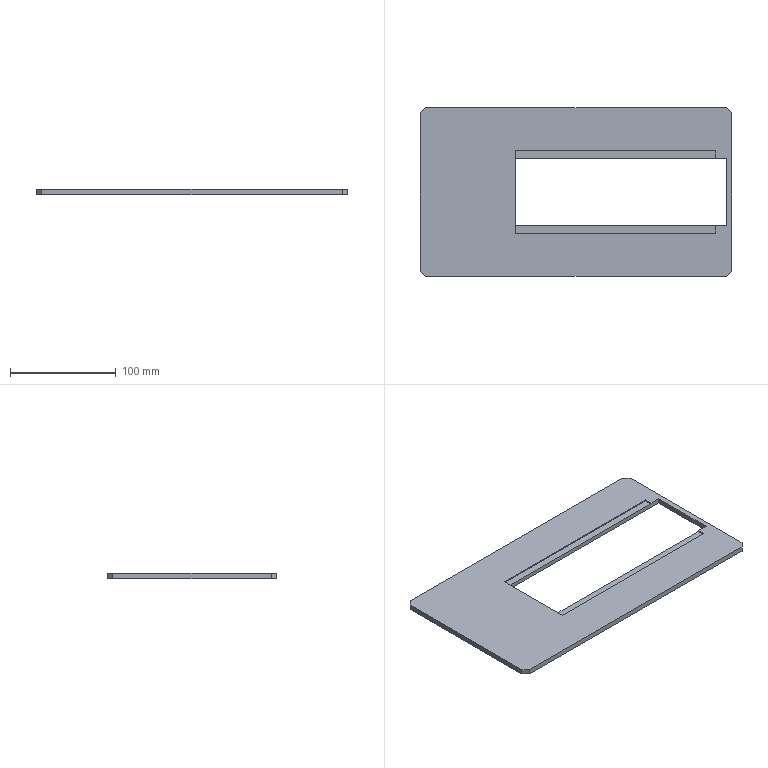Component | SolidWorks | 2023-12-12-25-1 | 1 solid | 38 faces | box 295 x 160 x 5 mm | volume 166969 mm3 | plane 26 | cylinder 12 | commonest cylinder face diameters 15 x12 | material S45C
build123d program:
from build123d import *

# Parameters (mm, degrees)
SKETCH1_2_W          = 200
SKETCH1_2_H          = 64
BOSS_EXTRUDE1_DEPTH  = 5
SKETCH3_R            = 7.5
CUT_EXTRUDE2_DEPTH   = 2
CHAMFER2_SIZE        = 5
SKETCH4_W            = 25
SKETCH4_H            = 160
CUT_EXTRUDE3_DEPTH   = 10
CHAMFER3_SIZE        = 5
SKETCH1_W            = 190
SKETCH1_H            = 8
RAILSEATREBATE_DEPTH = 1


with BuildPart() as part:
    # Sketch1_2 → Boss-Extrude1 (new body)
    with BuildSketch(Plane.XY):
        Polygon((0, 0), (320, 0), (320, 18), (320, 160), (0, 160), align=None)
        with Locations((130, 80)):
            Rectangle(SKETCH1_2_W, SKETCH1_2_H, mode=Mode.SUBTRACT)
    extrude(amount=BOSS_EXTRUDE1_DEPTH)

    # Sketch3 → Cut-Extrude2 (cut)
    with BuildSketch(Plane(origin=(0, 0, 0), x_dir=(-1, 0, 0), z_dir=(0, 0, -1))):
        with Locations((-305, 150)):
            Circle(SKETCH3_R)
        with Locations((-105, 150)):
            Circle(SKETCH3_R)
        with Locations((-40, 150)):
            Circle(SKETCH3_R)
        with Locations(Location((-40, 10, 0), (0, 0, 180))):
            Circle(SKETCH3_R)
        with Locations(Location((-105, 10, 0), (0, 0, 180))):
            Circle(SKETCH3_R)
        with Locations(Location((-305, 10, 0), (0, 0, 180))):
            Circle(SKETCH3_R)
    extrude(amount=-CUT_EXTRUDE2_DEPTH, mode=Mode.SUBTRACT)

    # Chamfer2
    chamfer2_edges = [part.edges().sort_by_distance(p)[0] for p in [
        (0, 160, 2.5),
        (320, 160, 2.5),
        (320, 0, 2.5),
        (0, 0, 2.5),
    ]]
    chamfer(chamfer2_edges, length=CHAMFER2_SIZE)

    # Sketch4 → Cut-Extrude3 (cut)
    with BuildSketch(Plane(origin=(0, 0, 0), x_dir=(-1, 0, 0), z_dir=(0, 0, -1))):
        with Locations((-12.5, 80)):
            Rectangle(SKETCH4_W, SKETCH4_H)
    extrude(amount=-CUT_EXTRUDE3_DEPTH, mode=Mode.SUBTRACT)

    # Chamfer3
    chamfer3_edges = [part.edges().sort_by_distance(p)[0] for p in [
        (25, 0, 2.5),
        (25, 160, 2.5),
    ]]
    chamfer(chamfer3_edges, length=CHAMFER3_SIZE)

    # Sketch1 → RailSeatRebate (cut)
    with BuildSketch(Plane.XY.offset(5)):
        with Locations((135, 45)):
            Rectangle(SKETCH1_W, SKETCH1_H)
        with Locations((135, 115)):
            Rectangle(SKETCH1_W, SKETCH1_H)
    extrude(amount=-RAILSEATREBATE_DEPTH, mode=Mode.SUBTRACT)


solid = part.part

# Placed as in the assembly
solid = solid.moved(Location((131.222, 77.133, 79), (0, 0, 180)))
STEP:
#1=COLOUR_RGB('',0.7922,0.8196,0.9333);
#2=FILL_AREA_STYLE_COLOUR('',#1);
#3=FILL_AREA_STYLE('',(#2));
#4=SURFACE_STYLE_FILL_AREA(#3);
#5=SURFACE_SIDE_STYLE('',(#4));
#6=SURFACE_STYLE_USAGE(.BOTH.,#5);
#7=PRESENTATION_STYLE_ASSIGNMENT((#6));
#8=CARTESIAN_POINT('',(3.296,-2.869,3.189));
#9=VERTEX_POINT('',#8);
#10=CARTESIAN_POINT('',(3.887,-2.869,3.189));
#11=VERTEX_POINT('',#10);
#12=CARTESIAN_POINT('',(3.591,-2.869,3.189));
#13=DIRECTION('',(0.,0.,-1.));
#14=DIRECTION('',(1.,0.,0.));
#15=AXIS2_PLACEMENT_3D('',#12,#13,#14);
#16=CIRCLE('',#15,0.2953);
#17=EDGE_CURVE('',#9,#11,#16,.T.);
#18=ORIENTED_EDGE('',*,*,#17,.F.);
#19=CARTESIAN_POINT('',(3.296,-2.869,3.11));
#20=VERTEX_POINT('',#19);
#21=CARTESIAN_POINT('',(3.296,-2.869,3.189));
#22=DIRECTION('',(0.,0.,-1.));
#23=VECTOR('',#22,39.37);
#24=LINE('',#21,#23);
#25=EDGE_CURVE('',#9,#20,#24,.T.);
#26=ORIENTED_EDGE('',*,*,#25,.T.);
#27=CARTESIAN_POINT('',(3.887,-2.869,3.11));
#28=VERTEX_POINT('',#27);
#29=CARTESIAN_POINT('',(3.591,-2.869,3.11));
#30=DIRECTION('',(0.,0.,-1.));
#31=DIRECTION('',(1.,0.,0.));
#32=AXIS2_PLACEMENT_3D('',#29,#30,#31);
#33=CIRCLE('',#32,0.2953);
#34=EDGE_CURVE('',#20,#28,#33,.T.);
#35=ORIENTED_EDGE('',*,*,#34,.T.);
#36=CARTESIAN_POINT('',(3.887,-2.869,3.189));
#37=DIRECTION('',(0.,0.,-1.));
#38=VECTOR('',#37,39.37);
#39=LINE('',#36,#38);
#40=EDGE_CURVE('',#11,#28,#39,.T.);
#41=ORIENTED_EDGE('',*,*,#40,.F.);
#42=EDGE_LOOP('',(#18,#26,#35,#41));
#43=FACE_OUTER_BOUND('',#42,.T.);
#44=CARTESIAN_POINT('',(3.591,-2.869,3.189));
#45=DIRECTION('',(0.,0.,-1.));
#46=DIRECTION('',(1.,0.,0.));
#47=AXIS2_PLACEMENT_3D('',#44,#45,#46);
#48=CYLINDRICAL_SURFACE('',#47,0.2953);
#49=ADVANCED_FACE('',(#43),#48,.F.);
#50=CARTESIAN_POINT('',(-7.137,-2.869,3.189));
#51=VERTEX_POINT('',#50);
#52=CARTESIAN_POINT('',(-6.546,-2.869,3.189));
#53=VERTEX_POINT('',#52);
#54=CARTESIAN_POINT('',(-6.842,-2.869,3.189));
#55=DIRECTION('',(0.,0.,-1.));
#56=DIRECTION('',(1.,0.,0.));
#57=AXIS2_PLACEMENT_3D('',#54,#55,#56);
#58=CIRCLE('',#57,0.2953);
#59=EDGE_CURVE('',#51,#53,#58,.T.);
#60=ORIENTED_EDGE('',*,*,#59,.F.);
#61=CARTESIAN_POINT('',(-7.137,-2.869,3.11));
#62=VERTEX_POINT('',#61);
#63=CARTESIAN_POINT('',(-7.137,-2.869,3.189));
#64=DIRECTION('',(0.,0.,-1.));
#65=VECTOR('',#64,39.37);
#66=LINE('',#63,#65);
#67=EDGE_CURVE('',#51,#62,#66,.T.);
#68=ORIENTED_EDGE('',*,*,#67,.T.);
#69=CARTESIAN_POINT('',(-6.546,-2.869,3.11));
#70=VERTEX_POINT('',#69);
#71=CARTESIAN_POINT('',(-6.842,-2.869,3.11));
#72=DIRECTION('',(0.,0.,-1.));
#73=DIRECTION('',(1.,0.,0.));
#74=AXIS2_PLACEMENT_3D('',#71,#72,#73);
#75=CIRCLE('',#74,0.2953);
#76=EDGE_CURVE('',#62,#70,#75,.T.);
#77=ORIENTED_EDGE('',*,*,#76,.T.);
#78=CARTESIAN_POINT('',(-6.546,-2.869,3.189));
#79=DIRECTION('',(0.,0.,-1.));
#80=VECTOR('',#79,39.37);
#81=LINE('',#78,#80);
#82=EDGE_CURVE('',#53,#70,#81,.T.);
#83=ORIENTED_EDGE('',*,*,#82,.F.);
#84=EDGE_LOOP('',(#60,#68,#77,#83));
#85=FACE_OUTER_BOUND('',#84,.T.);
#86=CARTESIAN_POINT('',(-6.842,-2.869,3.189));
#87=DIRECTION('',(0.,0.,-1.));
#88=DIRECTION('',(1.,0.,0.));
#89=AXIS2_PLACEMENT_3D('',#86,#87,#88);
#90=CYLINDRICAL_SURFACE('',#89,0.2953);
#91=ADVANCED_FACE('',(#85),#90,.F.);
#92=CARTESIAN_POINT('',(3.296,2.643,3.189));
#93=VERTEX_POINT('',#92);
#94=CARTESIAN_POINT('',(3.887,2.643,3.189));
#95=VERTEX_POINT('',#94);
#96=CARTESIAN_POINT('',(3.591,2.643,3.189));
#97=DIRECTION('',(0.,0.,-1.));
#98=DIRECTION('',(-1.,0.,0.));
#99=AXIS2_PLACEMENT_3D('',#96,#97,#98);
#100=CIRCLE('',#99,0.2953);
#101=EDGE_CURVE('',#93,#95,#100,.T.);
#102=ORIENTED_EDGE('',*,*,#101,.F.);
#103=CARTESIAN_POINT('',(3.296,2.643,3.11));
#104=VERTEX_POINT('',#103);
#105=CARTESIAN_POINT('',(3.296,2.643,3.189));
#106=DIRECTION('',(0.,0.,-1.));
#107=VECTOR('',#106,39.37);
#108=LINE('',#105,#107);
#109=EDGE_CURVE('',#93,#104,#108,.T.);
#110=ORIENTED_EDGE('',*,*,#109,.T.);
#111=CARTESIAN_POINT('',(3.887,2.643,3.11));
#112=VERTEX_POINT('',#111);
#113=CARTESIAN_POINT('',(3.591,2.643,3.11));
#114=DIRECTION('',(0.,0.,-1.));
#115=DIRECTION('',(-1.,0.,0.));
#116=AXIS2_PLACEMENT_3D('',#113,#114,#115);
#117=CIRCLE('',#116,0.2953);
#118=EDGE_CURVE('',#104,#112,#117,.T.);
#119=ORIENTED_EDGE('',*,*,#118,.T.);
#120=CARTESIAN_POINT('',(3.887,2.643,3.189));
#121=DIRECTION('',(0.,0.,-1.));
#122=VECTOR('',#121,39.37);
#123=LINE('',#120,#122);
#124=EDGE_CURVE('',#95,#112,#123,.T.);
#125=ORIENTED_EDGE('',*,*,#124,.F.);
#126=EDGE_LOOP('',(#102,#110,#119,#125));
#127=FACE_OUTER_BOUND('',#126,.T.);
#128=CARTESIAN_POINT('',(3.591,2.643,3.189));
#129=DIRECTION('',(0.,0.,-1.));
#130=DIRECTION('',(1.,0.,0.));
#131=AXIS2_PLACEMENT_3D('',#128,#129,#130);
#132=CYLINDRICAL_SURFACE('',#131,0.2953);
#133=ADVANCED_FACE('',(#127),#132,.F.);
#134=CARTESIAN_POINT('',(0.7371,2.643,3.189));
#135=VERTEX_POINT('',#134);
#136=CARTESIAN_POINT('',(1.328,2.643,3.189));
#137=VERTEX_POINT('',#136);
#138=CARTESIAN_POINT('',(1.032,2.643,3.189));
#139=DIRECTION('',(0.,0.,-1.));
#140=DIRECTION('',(-1.,0.,0.));
#141=AXIS2_PLACEMENT_3D('',#138,#139,#140);
#142=CIRCLE('',#141,0.2953);
#143=EDGE_CURVE('',#135,#137,#142,.T.);
#144=ORIENTED_EDGE('',*,*,#143,.F.);
#145=CARTESIAN_POINT('',(0.7371,2.643,3.11));
#146=VERTEX_POINT('',#145);
#147=CARTESIAN_POINT('',(0.7371,2.643,3.189));
#148=DIRECTION('',(0.,0.,-1.));
#149=VECTOR('',#148,39.37);
#150=LINE('',#147,#149);
#151=EDGE_CURVE('',#135,#146,#150,.T.);
#152=ORIENTED_EDGE('',*,*,#151,.T.);
#153=CARTESIAN_POINT('',(1.328,2.643,3.11));
#154=VERTEX_POINT('',#153);
#155=CARTESIAN_POINT('',(1.032,2.643,3.11));
#156=DIRECTION('',(0.,0.,-1.));
#157=DIRECTION('',(-1.,0.,0.));
#158=AXIS2_PLACEMENT_3D('',#155,#156,#157);
#159=CIRCLE('',#158,0.2953);
#160=EDGE_CURVE('',#146,#154,#159,.T.);
#161=ORIENTED_EDGE('',*,*,#160,.T.);
#162=CARTESIAN_POINT('',(1.328,2.643,3.189));
#163=DIRECTION('',(0.,0.,-1.));
#164=VECTOR('',#163,39.37);
#165=LINE('',#162,#164);
#166=EDGE_CURVE('',#137,#154,#165,.T.);
#167=ORIENTED_EDGE('',*,*,#166,.F.);
#168=EDGE_LOOP('',(#144,#152,#161,#167));
#169=FACE_OUTER_BOUND('',#168,.T.);
#170=CARTESIAN_POINT('',(1.032,2.643,3.189));
#171=DIRECTION('',(0.,0.,-1.));
#172=DIRECTION('',(1.,0.,0.));
#173=AXIS2_PLACEMENT_3D('',#170,#171,#172);
#174=CYLINDRICAL_SURFACE('',#173,0.2953);
#175=ADVANCED_FACE('',(#169),#174,.F.);
#176=CARTESIAN_POINT('',(-7.137,2.643,3.189));
#177=VERTEX_POINT('',#176);
#178=CARTESIAN_POINT('',(-6.546,2.643,3.189));
#179=VERTEX_POINT('',#178);
#180=CARTESIAN_POINT('',(-6.842,2.643,3.189));
#181=DIRECTION('',(0.,0.,-1.));
#182=DIRECTION('',(-1.,0.,0.));
#183=AXIS2_PLACEMENT_3D('',#180,#181,#182);
#184=CIRCLE('',#183,0.2953);
#185=EDGE_CURVE('',#177,#179,#184,.T.);
#186=ORIENTED_EDGE('',*,*,#185,.F.);
#187=CARTESIAN_POINT('',(-7.137,2.643,3.11));
#188=VERTEX_POINT('',#187);
#189=CARTESIAN_POINT('',(-7.137,2.643,3.189));
#190=DIRECTION('',(0.,0.,-1.));
#191=VECTOR('',#190,39.37);
#192=LINE('',#189,#191);
#193=EDGE_CURVE('',#177,#188,#192,.T.);
#194=ORIENTED_EDGE('',*,*,#193,.T.);
#195=CARTESIAN_POINT('',(-6.546,2.643,3.11));
#196=VERTEX_POINT('',#195);
#197=CARTESIAN_POINT('',(-6.842,2.643,3.11));
#198=DIRECTION('',(0.,0.,-1.));
#199=DIRECTION('',(-1.,0.,0.));
#200=AXIS2_PLACEMENT_3D('',#197,#198,#199);
#201=CIRCLE('',#200,0.2953);
#202=EDGE_CURVE('',#188,#196,#201,.T.);
#203=ORIENTED_EDGE('',*,*,#202,.T.);
#204=CARTESIAN_POINT('',(-6.546,2.643,3.189));
#205=DIRECTION('',(0.,0.,-1.));
#206=VECTOR('',#205,39.37);
#207=LINE('',#204,#206);
#208=EDGE_CURVE('',#179,#196,#207,.T.);
#209=ORIENTED_EDGE('',*,*,#208,.F.);
#210=EDGE_LOOP('',(#186,#194,#203,#209));
#211=FACE_OUTER_BOUND('',#210,.T.);
#212=CARTESIAN_POINT('',(-6.842,2.643,3.189));
#213=DIRECTION('',(0.,0.,-1.));
#214=DIRECTION('',(1.,0.,0.));
#215=AXIS2_PLACEMENT_3D('',#212,#213,#214);
#216=CYLINDRICAL_SURFACE('',#215,0.2953);
#217=ADVANCED_FACE('',(#211),#216,.F.);
#218=CARTESIAN_POINT('',(0.7371,-2.869,3.189));
#219=VERTEX_POINT('',#218);
#220=CARTESIAN_POINT('',(1.328,-2.869,3.189));
#221=VERTEX_POINT('',#220);
#222=CARTESIAN_POINT('',(1.032,-2.869,3.189));
#223=DIRECTION('',(0.,0.,-1.));
#224=DIRECTION('',(1.,0.,0.));
#225=AXIS2_PLACEMENT_3D('',#222,#223,#224);
#226=CIRCLE('',#225,0.2953);
#227=EDGE_CURVE('',#219,#221,#226,.T.);
#228=ORIENTED_EDGE('',*,*,#227,.F.);
#229=CARTESIAN_POINT('',(0.7371,-2.869,3.11));
#230=VERTEX_POINT('',#229);
#231=CARTESIAN_POINT('',(0.7371,-2.869,3.189));
#232=DIRECTION('',(0.,0.,-1.));
#233=VECTOR('',#232,39.37);
#234=LINE('',#231,#233);
#235=EDGE_CURVE('',#219,#230,#234,.T.);
#236=ORIENTED_EDGE('',*,*,#235,.T.);
#237=CARTESIAN_POINT('',(1.328,-2.869,3.11));
#238=VERTEX_POINT('',#237);
#239=CARTESIAN_POINT('',(1.032,-2.869,3.11));
#240=DIRECTION('',(0.,0.,-1.));
#241=DIRECTION('',(1.,0.,0.));
#242=AXIS2_PLACEMENT_3D('',#239,#240,#241);
#243=CIRCLE('',#242,0.2953);
#244=EDGE_CURVE('',#230,#238,#243,.T.);
#245=ORIENTED_EDGE('',*,*,#244,.T.);
#246=CARTESIAN_POINT('',(1.328,-2.869,3.189));
#247=DIRECTION('',(0.,0.,-1.));
#248=VECTOR('',#247,39.37);
#249=LINE('',#246,#248);
#250=EDGE_CURVE('',#221,#238,#249,.T.);
#251=ORIENTED_EDGE('',*,*,#250,.F.);
#252=EDGE_LOOP('',(#228,#236,#245,#251));
#253=FACE_OUTER_BOUND('',#252,.T.);
#254=CARTESIAN_POINT('',(1.032,-2.869,3.189));
#255=DIRECTION('',(0.,0.,-1.));
#256=DIRECTION('',(1.,0.,0.));
#257=AXIS2_PLACEMENT_3D('',#254,#255,#256);
#258=CYLINDRICAL_SURFACE('',#257,0.2953);
#259=ADVANCED_FACE('',(#253),#258,.F.);
#260=CARTESIAN_POINT('',(-7.235,-3.262,3.307));
#261=VERTEX_POINT('',#260);
#262=CARTESIAN_POINT('',(3.985,-3.262,3.307));
#263=VERTEX_POINT('',#262);
#264=CARTESIAN_POINT('',(5.166,-3.262,3.307));
#265=DIRECTION('',(1.,0.,0.));
#266=VECTOR('',#265,39.37);
#267=LINE('',#264,#266);
#268=EDGE_CURVE('',#261,#263,#267,.T.);
#269=ORIENTED_EDGE('',*,*,#268,.T.);
#270=CARTESIAN_POINT('',(4.182,-3.066,3.307));
#271=VERTEX_POINT('',#270);
#272=CARTESIAN_POINT('',(4.182,-3.066,3.307));
#273=DIRECTION('',(0.7071,0.7071,0.));
#274=VECTOR('',#273,39.37);
#275=LINE('',#272,#274);
#276=EDGE_CURVE('',#263,#271,#275,.T.);
#277=ORIENTED_EDGE('',*,*,#276,.T.);
#278=CARTESIAN_POINT('',(4.182,2.84,3.307));
#279=VERTEX_POINT('',#278);
#280=CARTESIAN_POINT('',(4.182,3.037,3.307));
#281=DIRECTION('',(0.,1.,0.));
#282=VECTOR('',#281,39.37);
#283=LINE('',#280,#282);
#284=EDGE_CURVE('',#271,#279,#283,.T.);
#285=ORIENTED_EDGE('',*,*,#284,.T.);
#286=CARTESIAN_POINT('',(3.985,3.037,3.307));
#287=VERTEX_POINT('',#286);
#288=CARTESIAN_POINT('',(3.985,3.037,3.307));
#289=DIRECTION('',(-0.7071,0.7071,0.));
#290=VECTOR('',#289,39.37);
#291=LINE('',#288,#290);
#292=EDGE_CURVE('',#279,#287,#291,.T.);
#293=ORIENTED_EDGE('',*,*,#292,.T.);
#294=CARTESIAN_POINT('',(-7.235,3.037,3.307));
#295=VERTEX_POINT('',#294);
#296=CARTESIAN_POINT('',(5.166,3.037,3.307));
#297=DIRECTION('',(-1.,0.,-0.));
#298=VECTOR('',#297,39.37);
#299=LINE('',#296,#298);
#300=EDGE_CURVE('',#287,#295,#299,.T.);
#301=ORIENTED_EDGE('',*,*,#300,.T.);
#302=CARTESIAN_POINT('',(-7.432,2.84,3.307));
#303=VERTEX_POINT('',#302);
#304=CARTESIAN_POINT('',(-7.432,2.84,3.307));
#305=DIRECTION('',(-0.7071,-0.7071,-0.));
#306=VECTOR('',#305,39.37);
#307=LINE('',#304,#306);
#308=EDGE_CURVE('',#295,#303,#307,.T.);
#309=ORIENTED_EDGE('',*,*,#308,.T.);
#310=CARTESIAN_POINT('',(-7.432,-3.066,3.307));
#311=VERTEX_POINT('',#310);
#312=CARTESIAN_POINT('',(-7.432,3.037,3.307));
#313=DIRECTION('',(-0.,-1.,-0.));
#314=VECTOR('',#313,39.37);
#315=LINE('',#312,#314);
#316=EDGE_CURVE('',#303,#311,#315,.T.);
#317=ORIENTED_EDGE('',*,*,#316,.T.);
#318=CARTESIAN_POINT('',(-7.235,-3.262,3.307));
#319=DIRECTION('',(0.7071,-0.7071,-0.));
#320=VECTOR('',#319,39.37);
#321=LINE('',#318,#320);
#322=EDGE_CURVE('',#311,#261,#321,.T.);
#323=ORIENTED_EDGE('',*,*,#322,.T.);
#324=EDGE_LOOP('',(#269,#277,#285,#293,#301,#309,#317,#323));
#325=FACE_OUTER_BOUND('',#324,.T.);
#326=CARTESIAN_POINT('',(3.591,1.147,3.307));
#327=VERTEX_POINT('',#326);
#328=CARTESIAN_POINT('',(3.591,1.423,3.307));
#329=VERTEX_POINT('',#328);
#330=CARTESIAN_POINT('',(3.591,1.423,3.307));
#331=DIRECTION('',(0.,1.,0.));
#332=VECTOR('',#331,39.37);
#333=LINE('',#330,#332);
#334=EDGE_CURVE('',#327,#329,#333,.T.);
#335=ORIENTED_EDGE('',*,*,#334,.F.);
#336=CARTESIAN_POINT('',(3.985,1.147,3.307));
#337=VERTEX_POINT('',#336);
#338=CARTESIAN_POINT('',(3.985,1.147,3.307));
#339=DIRECTION('',(-1.,0.,-0.));
#340=VECTOR('',#339,39.37);
#341=LINE('',#338,#340);
#342=EDGE_CURVE('',#337,#327,#341,.T.);
#343=ORIENTED_EDGE('',*,*,#342,.F.);
#344=CARTESIAN_POINT('',(3.985,-1.373,3.307));
#345=VERTEX_POINT('',#344);
#346=CARTESIAN_POINT('',(3.985,1.147,3.307));
#347=DIRECTION('',(0.,1.,0.));
#348=VECTOR('',#347,39.37);
#349=LINE('',#346,#348);
#350=EDGE_CURVE('',#345,#337,#349,.T.);
#351=ORIENTED_EDGE('',*,*,#350,.F.);
#352=CARTESIAN_POINT('',(3.591,-1.373,3.307));
#353=VERTEX_POINT('',#352);
#354=CARTESIAN_POINT('',(3.985,-1.373,3.307));
#355=DIRECTION('',(1.,-0.,0.));
#356=VECTOR('',#355,39.37);
#357=LINE('',#354,#356);
#358=EDGE_CURVE('',#353,#345,#357,.T.);
#359=ORIENTED_EDGE('',*,*,#358,.F.);
#360=CARTESIAN_POINT('',(3.591,-1.648,3.307));
#361=VERTEX_POINT('',#360);
#362=CARTESIAN_POINT('',(3.591,-1.333,3.307));
#363=DIRECTION('',(0.,1.,0.));
#364=VECTOR('',#363,39.37);
#365=LINE('',#362,#364);
#366=EDGE_CURVE('',#361,#353,#365,.T.);
#367=ORIENTED_EDGE('',*,*,#366,.F.);
#368=CARTESIAN_POINT('',(-3.889,-1.648,3.307));
#369=VERTEX_POINT('',#368);
#370=CARTESIAN_POINT('',(3.591,-1.648,3.307));
#371=DIRECTION('',(1.,-0.,0.));
#372=VECTOR('',#371,39.37);
#373=LINE('',#370,#372);
#374=EDGE_CURVE('',#369,#361,#373,.T.);
#375=ORIENTED_EDGE('',*,*,#374,.F.);
#376=CARTESIAN_POINT('',(-3.889,1.423,3.307));
#377=VERTEX_POINT('',#376);
#378=CARTESIAN_POINT('',(-3.889,-1.373,3.307));
#379=DIRECTION('',(-0.,-1.,-0.));
#380=VECTOR('',#379,39.37);
#381=LINE('',#378,#380);
#382=EDGE_CURVE('',#377,#369,#381,.T.);
#383=ORIENTED_EDGE('',*,*,#382,.F.);
#384=CARTESIAN_POINT('',(3.591,1.423,3.307));
#385=DIRECTION('',(-1.,0.,-0.));
#386=VECTOR('',#385,39.37);
#387=LINE('',#384,#386);
#388=EDGE_CURVE('',#329,#377,#387,.T.);
#389=ORIENTED_EDGE('',*,*,#388,.F.);
#390=EDGE_LOOP('',(#335,#343,#351,#359,#367,#375,#383,#389));
#391=FACE_BOUND('',#390,.T.);
#392=CARTESIAN_POINT('',(5.166,3.037,3.307));
#393=DIRECTION('',(0.,0.,-1.));
#394=DIRECTION('',(1.,-0.,0.));
#395=AXIS2_PLACEMENT_3D('',#392,#393,#394);
#396=PLANE('',#395);
#397=ADVANCED_FACE('',(#325,#391),#396,.F.);
#398=CARTESIAN_POINT('',(4.182,-3.066,3.11));
#399=VERTEX_POINT('',#398);
#400=CARTESIAN_POINT('',(4.182,2.84,3.11));
#401=VERTEX_POINT('',#400);
#402=CARTESIAN_POINT('',(4.182,-3.262,3.11));
#403=DIRECTION('',(0.,1.,0.));
#404=VECTOR('',#403,39.37);
#405=LINE('',#402,#404);
#406=EDGE_CURVE('',#399,#401,#405,.T.);
#407=ORIENTED_EDGE('',*,*,#406,.F.);
#408=CARTESIAN_POINT('',(3.985,-3.262,3.11));
#409=VERTEX_POINT('',#408);
#410=CARTESIAN_POINT('',(7.725,0.4777,3.11));
#411=DIRECTION('',(-0.7071,-0.7071,-0.));
#412=VECTOR('',#411,39.37);
#413=LINE('',#410,#412);
#414=EDGE_CURVE('',#399,#409,#413,.T.);
#415=ORIENTED_EDGE('',*,*,#414,.T.);
#416=CARTESIAN_POINT('',(-7.235,-3.262,3.11));
#417=VERTEX_POINT('',#416);
#418=CARTESIAN_POINT('',(5.166,-3.262,3.11));
#419=DIRECTION('',(1.,0.,0.));
#420=VECTOR('',#419,39.37);
#421=LINE('',#418,#420);
#422=EDGE_CURVE('',#417,#409,#421,.T.);
#423=ORIENTED_EDGE('',*,*,#422,.F.);
#424=CARTESIAN_POINT('',(-7.432,-3.066,3.11));
#425=VERTEX_POINT('',#424);
#426=CARTESIAN_POINT('',(-4.184,-6.314,3.11));
#427=DIRECTION('',(-0.7071,0.7071,0.));
#428=VECTOR('',#427,39.37);
#429=LINE('',#426,#428);
#430=EDGE_CURVE('',#417,#425,#429,.T.);
#431=ORIENTED_EDGE('',*,*,#430,.T.);
#432=CARTESIAN_POINT('',(-7.432,2.84,3.11));
#433=VERTEX_POINT('',#432);
#434=CARTESIAN_POINT('',(-7.432,-3.262,3.11));
#435=DIRECTION('',(0.,-1.,-0.));
#436=VECTOR('',#435,39.37);
#437=LINE('',#434,#436);
#438=EDGE_CURVE('',#433,#425,#437,.T.);
#439=ORIENTED_EDGE('',*,*,#438,.F.);
#440=CARTESIAN_POINT('',(-7.235,3.037,3.11));
#441=VERTEX_POINT('',#440);
#442=CARTESIAN_POINT('',(-1.035,9.238,3.11));
#443=DIRECTION('',(0.7071,0.7071,0.));
#444=VECTOR('',#443,39.37);
#445=LINE('',#442,#444);
#446=EDGE_CURVE('',#433,#441,#445,.T.);
#447=ORIENTED_EDGE('',*,*,#446,.T.);
#448=CARTESIAN_POINT('',(3.985,3.037,3.11));
#449=VERTEX_POINT('',#448);
#450=CARTESIAN_POINT('',(5.166,3.037,3.11));
#451=DIRECTION('',(-1.,0.,-0.));
#452=VECTOR('',#451,39.37);
#453=LINE('',#450,#452);
#454=EDGE_CURVE('',#449,#441,#453,.T.);
#455=ORIENTED_EDGE('',*,*,#454,.F.);
#456=CARTESIAN_POINT('',(4.576,2.446,3.11));
#457=DIRECTION('',(0.7071,-0.7071,-0.));
#458=VECTOR('',#457,39.37);
#459=LINE('',#456,#458);
#460=EDGE_CURVE('',#449,#401,#459,.T.);
#461=ORIENTED_EDGE('',*,*,#460,.T.);
#462=EDGE_LOOP('',(#407,#415,#423,#431,#439,#447,#455,#461));
#463=FACE_OUTER_BOUND('',#462,.T.);
#464=CARTESIAN_POINT('',(3.591,-2.869,3.11));
#465=DIRECTION('',(0.,0.,-1.));
#466=DIRECTION('',(1.,0.,0.));
#467=AXIS2_PLACEMENT_3D('',#464,#465,#466);
#468=CIRCLE('',#467,0.2953);
#469=EDGE_CURVE('',#28,#20,#468,.T.);
#470=ORIENTED_EDGE('',*,*,#469,.F.);
#471=ORIENTED_EDGE('',*,*,#34,.F.);
#472=EDGE_LOOP('',(#470,#471));
#473=FACE_BOUND('',#472,.T.);
#474=CARTESIAN_POINT('',(-6.842,-2.869,3.11));
#475=DIRECTION('',(0.,0.,-1.));
#476=DIRECTION('',(1.,0.,0.));
#477=AXIS2_PLACEMENT_3D('',#474,#475,#476);
#478=CIRCLE('',#477,0.2953);
#479=EDGE_CURVE('',#70,#62,#478,.T.);
#480=ORIENTED_EDGE('',*,*,#479,.F.);
#481=ORIENTED_EDGE('',*,*,#76,.F.);
#482=EDGE_LOOP('',(#480,#481));
#483=FACE_BOUND('',#482,.T.);
#484=CARTESIAN_POINT('',(3.591,2.643,3.11));
#485=DIRECTION('',(0.,0.,-1.));
#486=DIRECTION('',(-1.,0.,0.));
#487=AXIS2_PLACEMENT_3D('',#484,#485,#486);
#488=CIRCLE('',#487,0.2953);
#489=EDGE_CURVE('',#112,#104,#488,.T.);
#490=ORIENTED_EDGE('',*,*,#489,.F.);
#491=ORIENTED_EDGE('',*,*,#118,.F.);
#492=EDGE_LOOP('',(#490,#491));
#493=FACE_BOUND('',#492,.T.);
#494=CARTESIAN_POINT('',(1.032,2.643,3.11));
#495=DIRECTION('',(0.,0.,-1.));
#496=DIRECTION('',(-1.,0.,0.));
#497=AXIS2_PLACEMENT_3D('',#494,#495,#496);
#498=CIRCLE('',#497,0.2953);
#499=EDGE_CURVE('',#154,#146,#498,.T.);
#500=ORIENTED_EDGE('',*,*,#499,.F.);
#501=ORIENTED_EDGE('',*,*,#160,.F.);
#502=EDGE_LOOP('',(#500,#501));
#503=FACE_BOUND('',#502,.T.);
#504=CARTESIAN_POINT('',(-6.842,2.643,3.11));
#505=DIRECTION('',(0.,0.,-1.));
#506=DIRECTION('',(-1.,0.,0.));
#507=AXIS2_PLACEMENT_3D('',#504,#505,#506);
#508=CIRCLE('',#507,0.2953);
#509=EDGE_CURVE('',#196,#188,#508,.T.);
#510=ORIENTED_EDGE('',*,*,#509,.F.);
#511=ORIENTED_EDGE('',*,*,#202,.F.);
#512=EDGE_LOOP('',(#510,#511));
#513=FACE_BOUND('',#512,.T.);
#514=CARTESIAN_POINT('',(1.032,-2.869,3.11));
#515=DIRECTION('',(0.,0.,-1.));
#516=DIRECTION('',(1.,0.,0.));
#517=AXIS2_PLACEMENT_3D('',#514,#515,#516);
#518=CIRCLE('',#517,0.2953);
#519=EDGE_CURVE('',#238,#230,#518,.T.);
#520=ORIENTED_EDGE('',*,*,#519,.F.);
#521=ORIENTED_EDGE('',*,*,#244,.F.);
#522=EDGE_LOOP('',(#520,#521));
#523=FACE_BOUND('',#522,.T.);
#524=CARTESIAN_POINT('',(-3.889,-1.373,3.11));
#525=VERTEX_POINT('',#524);
#526=CARTESIAN_POINT('',(3.985,-1.373,3.11));
#527=VERTEX_POINT('',#526);
#528=CARTESIAN_POINT('',(3.985,-1.373,3.11));
#529=DIRECTION('',(1.,-0.,0.));
#530=VECTOR('',#529,39.37);
#531=LINE('',#528,#530);
#532=EDGE_CURVE('',#525,#527,#531,.T.);
#533=ORIENTED_EDGE('',*,*,#532,.T.);
#534=CARTESIAN_POINT('',(3.985,1.147,3.11));
#535=VERTEX_POINT('',#534);
#536=CARTESIAN_POINT('',(3.985,1.147,3.11));
#537=DIRECTION('',(0.,1.,0.));
#538=VECTOR('',#537,39.37);
#539=LINE('',#536,#538);
#540=EDGE_CURVE('',#527,#535,#539,.T.);
#541=ORIENTED_EDGE('',*,*,#540,.T.);
#542=CARTESIAN_POINT('',(-3.889,1.147,3.11));
#543=VERTEX_POINT('',#542);
#544=CARTESIAN_POINT('',(3.985,1.147,3.11));
#545=DIRECTION('',(-1.,0.,-0.));
#546=VECTOR('',#545,39.37);
#547=LINE('',#544,#546);
#548=EDGE_CURVE('',#535,#543,#547,.T.);
#549=ORIENTED_EDGE('',*,*,#548,.T.);
#550=CARTESIAN_POINT('',(-3.889,-1.373,3.11));
#551=DIRECTION('',(-0.,-1.,-0.));
#552=VECTOR('',#551,39.37);
#553=LINE('',#550,#552);
#554=EDGE_CURVE('',#543,#525,#553,.T.);
#555=ORIENTED_EDGE('',*,*,#554,.T.);
#556=EDGE_LOOP('',(#533,#541,#549,#555));
#557=FACE_BOUND('',#556,.T.);
#558=CARTESIAN_POINT('',(5.166,3.037,3.11));
#559=DIRECTION('',(0.,0.,-1.));
#560=DIRECTION('',(1.,-0.,0.));
#561=AXIS2_PLACEMENT_3D('',#558,#559,#560);
#562=PLANE('',#561);
#563=ADVANCED_FACE('',(#463,#473,#483,#493,#503,#513,#523,#557),#562,.T.);
#564=ORIENTED_EDGE('',*,*,#300,.F.);
#565=CARTESIAN_POINT('',(3.985,3.037,3.307));
#566=DIRECTION('',(0.,0.,-1.));
#567=VECTOR('',#566,39.37);
#568=LINE('',#565,#567);
#569=EDGE_CURVE('',#287,#449,#568,.T.);
#570=ORIENTED_EDGE('',*,*,#569,.T.);
#571=ORIENTED_EDGE('',*,*,#454,.T.);
#572=CARTESIAN_POINT('',(-7.235,3.037,3.307));
#573=DIRECTION('',(-0.,-0.,1.));
#574=VECTOR('',#573,39.37);
#575=LINE('',#572,#574);
#576=EDGE_CURVE('',#441,#295,#575,.T.);
#577=ORIENTED_EDGE('',*,*,#576,.T.);
#578=EDGE_LOOP('',(#564,#570,#571,#577));
#579=FACE_OUTER_BOUND('',#578,.T.);
#580=CARTESIAN_POINT('',(5.166,3.037,3.307));
#581=DIRECTION('',(-0.,-1.,-0.));
#582=DIRECTION('',(-0.,-0.,1.));
#583=AXIS2_PLACEMENT_3D('',#580,#581,#582);
#584=PLANE('',#583);
#585=ADVANCED_FACE('',(#579),#584,.F.);
#586=ORIENTED_EDGE('',*,*,#316,.F.);
#587=CARTESIAN_POINT('',(-7.432,2.84,3.307));
#588=DIRECTION('',(0.,0.,-1.));
#589=VECTOR('',#588,39.37);
#590=LINE('',#587,#589);
#591=EDGE_CURVE('',#303,#433,#590,.T.);
#592=ORIENTED_EDGE('',*,*,#591,.T.);
#593=ORIENTED_EDGE('',*,*,#438,.T.);
#594=CARTESIAN_POINT('',(-7.432,-3.066,3.307));
#595=DIRECTION('',(-0.,-0.,1.));
#596=VECTOR('',#595,39.37);
#597=LINE('',#594,#596);
#598=EDGE_CURVE('',#425,#311,#597,.T.);
#599=ORIENTED_EDGE('',*,*,#598,.T.);
#600=EDGE_LOOP('',(#586,#592,#593,#599));
#601=FACE_OUTER_BOUND('',#600,.T.);
#602=CARTESIAN_POINT('',(-7.432,-3.262,3.307));
#603=DIRECTION('',(1.,0.,0.));
#604=DIRECTION('',(-0.,1.,0.));
#605=AXIS2_PLACEMENT_3D('',#602,#603,#604);
#606=PLANE('',#605);
#607=ADVANCED_FACE('',(#601),#606,.F.);
#608=ORIENTED_EDGE('',*,*,#422,.T.);
#609=CARTESIAN_POINT('',(3.985,-3.262,3.307));
#610=DIRECTION('',(-0.,-0.,1.));
#611=VECTOR('',#610,39.37);
#612=LINE('',#609,#611);
#613=EDGE_CURVE('',#409,#263,#612,.T.);
#614=ORIENTED_EDGE('',*,*,#613,.T.);
#615=ORIENTED_EDGE('',*,*,#268,.F.);
#616=CARTESIAN_POINT('',(-7.235,-3.262,3.307));
#617=DIRECTION('',(0.,0.,-1.));
#618=VECTOR('',#617,39.37);
#619=LINE('',#616,#618);
#620=EDGE_CURVE('',#261,#417,#619,.T.);
#621=ORIENTED_EDGE('',*,*,#620,.T.);
#622=EDGE_LOOP('',(#608,#614,#615,#621));
#623=FACE_OUTER_BOUND('',#622,.T.);
#624=CARTESIAN_POINT('',(5.166,-3.262,3.307));
#625=DIRECTION('',(-0.,1.,0.));
#626=DIRECTION('',(-1.,-0.,-0.));
#627=AXIS2_PLACEMENT_3D('',#624,#625,#626);
#628=PLANE('',#627);
#629=ADVANCED_FACE('',(#623),#628,.F.);
#630=ORIENTED_EDGE('',*,*,#540,.F.);
#631=CARTESIAN_POINT('',(3.985,-1.373,3.307));
#632=DIRECTION('',(0.,0.,-1.));
#633=VECTOR('',#632,39.37);
#634=LINE('',#631,#633);
#635=EDGE_CURVE('',#345,#527,#634,.T.);
#636=ORIENTED_EDGE('',*,*,#635,.F.);
#637=ORIENTED_EDGE('',*,*,#350,.T.);
#638=CARTESIAN_POINT('',(3.985,1.147,3.307));
#639=DIRECTION('',(0.,0.,-1.));
#640=VECTOR('',#639,39.37);
#641=LINE('',#638,#640);
#642=EDGE_CURVE('',#337,#535,#641,.T.);
#643=ORIENTED_EDGE('',*,*,#642,.T.);
#644=EDGE_LOOP('',(#630,#636,#637,#643));
#645=FACE_OUTER_BOUND('',#644,.T.);
#646=CARTESIAN_POINT('',(3.985,1.147,3.307));
#647=DIRECTION('',(-1.,0.,-0.));
#648=DIRECTION('',(0.,0.,-1.));
#649=AXIS2_PLACEMENT_3D('',#646,#647,#648);
#650=PLANE('',#649);
#651=ADVANCED_FACE('',(#645),#650,.T.);
#652=CARTESIAN_POINT('',(3.591,1.147,3.268));
#653=VERTEX_POINT('',#652);
#654=CARTESIAN_POINT('',(3.591,1.147,3.307));
#655=DIRECTION('',(-0.,-0.,1.));
#656=VECTOR('',#655,39.37);
#657=LINE('',#654,#656);
#658=EDGE_CURVE('',#653,#327,#657,.T.);
#659=ORIENTED_EDGE('',*,*,#658,.F.);
#660=CARTESIAN_POINT('',(-3.889,1.147,3.268));
#661=VERTEX_POINT('',#660);
#662=CARTESIAN_POINT('',(3.985,1.147,3.268));
#663=DIRECTION('',(1.,-0.,0.));
#664=VECTOR('',#663,39.37);
#665=LINE('',#662,#664);
#666=EDGE_CURVE('',#661,#653,#665,.T.);
#667=ORIENTED_EDGE('',*,*,#666,.F.);
#668=CARTESIAN_POINT('',(-3.889,1.147,3.307));
#669=DIRECTION('',(0.,0.,-1.));
#670=VECTOR('',#669,39.37);
#671=LINE('',#668,#670);
#672=EDGE_CURVE('',#661,#543,#671,.T.);
#673=ORIENTED_EDGE('',*,*,#672,.T.);
#674=ORIENTED_EDGE('',*,*,#548,.F.);
#675=ORIENTED_EDGE('',*,*,#642,.F.);
#676=ORIENTED_EDGE('',*,*,#342,.T.);
#677=EDGE_LOOP('',(#659,#667,#673,#674,#675,#676));
#678=FACE_OUTER_BOUND('',#677,.T.);
#679=CARTESIAN_POINT('',(3.985,1.147,3.307));
#680=DIRECTION('',(-0.,-1.,-0.));
#681=DIRECTION('',(-0.,-0.,1.));
#682=AXIS2_PLACEMENT_3D('',#679,#680,#681);
#683=PLANE('',#682);
#684=ADVANCED_FACE('',(#678),#683,.T.);
#685=ORIENTED_EDGE('',*,*,#672,.F.);
#686=CARTESIAN_POINT('',(-3.889,1.423,3.268));
#687=VERTEX_POINT('',#686);
#688=CARTESIAN_POINT('',(-3.889,1.423,3.268));
#689=DIRECTION('',(-0.,-1.,-0.));
#690=VECTOR('',#689,39.37);
#691=LINE('',#688,#690);
#692=EDGE_CURVE('',#687,#661,#691,.T.);
#693=ORIENTED_EDGE('',*,*,#692,.F.);
#694=CARTESIAN_POINT('',(-3.889,1.423,3.268));
#695=DIRECTION('',(-0.,-0.,1.));
#696=VECTOR('',#695,39.37);
#697=LINE('',#694,#696);
#698=EDGE_CURVE('',#687,#377,#697,.T.);
#699=ORIENTED_EDGE('',*,*,#698,.T.);
#700=ORIENTED_EDGE('',*,*,#382,.T.);
#701=CARTESIAN_POINT('',(-3.889,-1.648,3.268));
#702=VERTEX_POINT('',#701);
#703=CARTESIAN_POINT('',(-3.889,-1.648,3.268));
#704=DIRECTION('',(-0.,-0.,1.));
#705=VECTOR('',#704,39.37);
#706=LINE('',#703,#705);
#707=EDGE_CURVE('',#702,#369,#706,.T.);
#708=ORIENTED_EDGE('',*,*,#707,.F.);
#709=CARTESIAN_POINT('',(-3.889,-1.373,3.268));
#710=VERTEX_POINT('',#709);
#711=CARTESIAN_POINT('',(-3.889,-1.333,3.268));
#712=DIRECTION('',(-0.,-1.,-0.));
#713=VECTOR('',#712,39.37);
#714=LINE('',#711,#713);
#715=EDGE_CURVE('',#710,#702,#714,.T.);
#716=ORIENTED_EDGE('',*,*,#715,.F.);
#717=CARTESIAN_POINT('',(-3.889,-1.373,3.307));
#718=DIRECTION('',(0.,0.,-1.));
#719=VECTOR('',#718,39.37);
#720=LINE('',#717,#719);
#721=EDGE_CURVE('',#710,#525,#720,.T.);
#722=ORIENTED_EDGE('',*,*,#721,.T.);
#723=ORIENTED_EDGE('',*,*,#554,.F.);
#724=EDGE_LOOP('',(#685,#693,#699,#700,#708,#716,#722,#723));
#725=FACE_OUTER_BOUND('',#724,.T.);
#726=CARTESIAN_POINT('',(-3.889,-1.373,3.307));
#727=DIRECTION('',(1.,-0.,0.));
#728=DIRECTION('',(-0.,-0.,1.));
#729=AXIS2_PLACEMENT_3D('',#726,#727,#728);
#730=PLANE('',#729);
#731=ADVANCED_FACE('',(#725),#730,.T.);
#732=CARTESIAN_POINT('',(3.591,-1.373,3.268));
#733=VERTEX_POINT('',#732);
#734=CARTESIAN_POINT('',(3.591,-1.373,3.307));
#735=DIRECTION('',(0.,0.,-1.));
#736=VECTOR('',#735,39.37);
#737=LINE('',#734,#736);
#738=EDGE_CURVE('',#353,#733,#737,.T.);
#739=ORIENTED_EDGE('',*,*,#738,.F.);
#740=ORIENTED_EDGE('',*,*,#358,.T.);
#741=ORIENTED_EDGE('',*,*,#635,.T.);
#742=ORIENTED_EDGE('',*,*,#532,.F.);
#743=ORIENTED_EDGE('',*,*,#721,.F.);
#744=CARTESIAN_POINT('',(3.985,-1.373,3.268));
#745=DIRECTION('',(-1.,0.,-0.));
#746=VECTOR('',#745,39.37);
#747=LINE('',#744,#746);
#748=EDGE_CURVE('',#733,#710,#747,.T.);
#749=ORIENTED_EDGE('',*,*,#748,.F.);
#750=EDGE_LOOP('',(#739,#740,#741,#742,#743,#749));
#751=FACE_OUTER_BOUND('',#750,.T.);
#752=CARTESIAN_POINT('',(3.985,-1.373,3.307));
#753=DIRECTION('',(0.,1.,0.));
#754=DIRECTION('',(0.,0.,-1.));
#755=AXIS2_PLACEMENT_3D('',#752,#753,#754);
#756=PLANE('',#755);
#757=ADVANCED_FACE('',(#751),#756,.T.);
#758=ORIENTED_EDGE('',*,*,#235,.F.);
#759=CARTESIAN_POINT('',(1.032,-2.869,3.189));
#760=DIRECTION('',(0.,0.,-1.));
#761=DIRECTION('',(1.,0.,0.));
#762=AXIS2_PLACEMENT_3D('',#759,#760,#761);
#763=CIRCLE('',#762,0.2953);
#764=EDGE_CURVE('',#221,#219,#763,.T.);
#765=ORIENTED_EDGE('',*,*,#764,.F.);
#766=ORIENTED_EDGE('',*,*,#250,.T.);
#767=ORIENTED_EDGE('',*,*,#519,.T.);
#768=EDGE_LOOP('',(#758,#765,#766,#767));
#769=FACE_OUTER_BOUND('',#768,.T.);
#770=CARTESIAN_POINT('',(1.032,-2.869,3.189));
#771=DIRECTION('',(0.,0.,-1.));
#772=DIRECTION('',(1.,0.,0.));
#773=AXIS2_PLACEMENT_3D('',#770,#771,#772);
#774=CYLINDRICAL_SURFACE('',#773,0.2953);
#775=ADVANCED_FACE('',(#769),#774,.F.);
#776=ORIENTED_EDGE('',*,*,#764,.T.);
#777=ORIENTED_EDGE('',*,*,#227,.T.);
#778=EDGE_LOOP('',(#776,#777));
#779=FACE_OUTER_BOUND('',#778,.T.);
#780=CARTESIAN_POINT('',(1.032,-2.869,3.189));
#781=DIRECTION('',(0.,0.,-1.));
#782=DIRECTION('',(1.,-0.,0.));
#783=AXIS2_PLACEMENT_3D('',#780,#781,#782);
#784=PLANE('',#783);
#785=ADVANCED_FACE('',(#779),#784,.T.);
#786=ORIENTED_EDGE('',*,*,#193,.F.);
#787=CARTESIAN_POINT('',(-6.842,2.643,3.189));
#788=DIRECTION('',(0.,0.,-1.));
#789=DIRECTION('',(-1.,0.,0.));
#790=AXIS2_PLACEMENT_3D('',#787,#788,#789);
#791=CIRCLE('',#790,0.2953);
#792=EDGE_CURVE('',#179,#177,#791,.T.);
#793=ORIENTED_EDGE('',*,*,#792,.F.);
#794=ORIENTED_EDGE('',*,*,#208,.T.);
#795=ORIENTED_EDGE('',*,*,#509,.T.);
#796=EDGE_LOOP('',(#786,#793,#794,#795));
#797=FACE_OUTER_BOUND('',#796,.T.);
#798=CARTESIAN_POINT('',(-6.842,2.643,3.189));
#799=DIRECTION('',(0.,0.,-1.));
#800=DIRECTION('',(1.,0.,0.));
#801=AXIS2_PLACEMENT_3D('',#798,#799,#800);
#802=CYLINDRICAL_SURFACE('',#801,0.2953);
#803=ADVANCED_FACE('',(#797),#802,.F.);
#804=ORIENTED_EDGE('',*,*,#792,.T.);
#805=ORIENTED_EDGE('',*,*,#185,.T.);
#806=EDGE_LOOP('',(#804,#805));
#807=FACE_OUTER_BOUND('',#806,.T.);
#808=CARTESIAN_POINT('',(-6.842,2.643,3.189));
#809=DIRECTION('',(-0.,-0.,1.));
#810=DIRECTION('',(-1.,0.,-0.));
#811=AXIS2_PLACEMENT_3D('',#808,#809,#810);
#812=PLANE('',#811);
#813=ADVANCED_FACE('',(#807),#812,.F.);
#814=ORIENTED_EDGE('',*,*,#151,.F.);
#815=CARTESIAN_POINT('',(1.032,2.643,3.189));
#816=DIRECTION('',(0.,0.,-1.));
#817=DIRECTION('',(-1.,0.,0.));
#818=AXIS2_PLACEMENT_3D('',#815,#816,#817);
#819=CIRCLE('',#818,0.2953);
#820=EDGE_CURVE('',#137,#135,#819,.T.);
#821=ORIENTED_EDGE('',*,*,#820,.F.);
#822=ORIENTED_EDGE('',*,*,#166,.T.);
#823=ORIENTED_EDGE('',*,*,#499,.T.);
#824=EDGE_LOOP('',(#814,#821,#822,#823));
#825=FACE_OUTER_BOUND('',#824,.T.);
#826=CARTESIAN_POINT('',(1.032,2.643,3.189));
#827=DIRECTION('',(0.,0.,-1.));
#828=DIRECTION('',(1.,0.,0.));
#829=AXIS2_PLACEMENT_3D('',#826,#827,#828);
#830=CYLINDRICAL_SURFACE('',#829,0.2953);
#831=ADVANCED_FACE('',(#825),#830,.F.);
#832=ORIENTED_EDGE('',*,*,#820,.T.);
#833=ORIENTED_EDGE('',*,*,#143,.T.);
#834=EDGE_LOOP('',(#832,#833));
#835=FACE_OUTER_BOUND('',#834,.T.);
#836=CARTESIAN_POINT('',(1.032,2.643,3.189));
#837=DIRECTION('',(-0.,-0.,1.));
#838=DIRECTION('',(-1.,0.,-0.));
#839=AXIS2_PLACEMENT_3D('',#836,#837,#838);
#840=PLANE('',#839);
#841=ADVANCED_FACE('',(#835),#840,.F.);
#842=ORIENTED_EDGE('',*,*,#109,.F.);
#843=CARTESIAN_POINT('',(3.591,2.643,3.189));
#844=DIRECTION('',(0.,0.,-1.));
#845=DIRECTION('',(-1.,0.,0.));
#846=AXIS2_PLACEMENT_3D('',#843,#844,#845);
#847=CIRCLE('',#846,0.2953);
#848=EDGE_CURVE('',#95,#93,#847,.T.);
#849=ORIENTED_EDGE('',*,*,#848,.F.);
#850=ORIENTED_EDGE('',*,*,#124,.T.);
#851=ORIENTED_EDGE('',*,*,#489,.T.);
#852=EDGE_LOOP('',(#842,#849,#850,#851));
#853=FACE_OUTER_BOUND('',#852,.T.);
#854=CARTESIAN_POINT('',(3.591,2.643,3.189));
#855=DIRECTION('',(0.,0.,-1.));
#856=DIRECTION('',(1.,0.,0.));
#857=AXIS2_PLACEMENT_3D('',#854,#855,#856);
#858=CYLINDRICAL_SURFACE('',#857,0.2953);
#859=ADVANCED_FACE('',(#853),#858,.F.);
#860=ORIENTED_EDGE('',*,*,#848,.T.);
#861=ORIENTED_EDGE('',*,*,#101,.T.);
#862=EDGE_LOOP('',(#860,#861));
#863=FACE_OUTER_BOUND('',#862,.T.);
#864=CARTESIAN_POINT('',(3.591,2.643,3.189));
#865=DIRECTION('',(-0.,-0.,1.));
#866=DIRECTION('',(-1.,0.,-0.));
#867=AXIS2_PLACEMENT_3D('',#864,#865,#866);
#868=PLANE('',#867);
#869=ADVANCED_FACE('',(#863),#868,.F.);
#870=ORIENTED_EDGE('',*,*,#67,.F.);
#871=CARTESIAN_POINT('',(-6.842,-2.869,3.189));
#872=DIRECTION('',(0.,0.,-1.));
#873=DIRECTION('',(1.,0.,0.));
#874=AXIS2_PLACEMENT_3D('',#871,#872,#873);
#875=CIRCLE('',#874,0.2953);
#876=EDGE_CURVE('',#53,#51,#875,.T.);
#877=ORIENTED_EDGE('',*,*,#876,.F.);
#878=ORIENTED_EDGE('',*,*,#82,.T.);
#879=ORIENTED_EDGE('',*,*,#479,.T.);
#880=EDGE_LOOP('',(#870,#877,#878,#879));
#881=FACE_OUTER_BOUND('',#880,.T.);
#882=CARTESIAN_POINT('',(-6.842,-2.869,3.189));
#883=DIRECTION('',(0.,0.,-1.));
#884=DIRECTION('',(1.,0.,0.));
#885=AXIS2_PLACEMENT_3D('',#882,#883,#884);
#886=CYLINDRICAL_SURFACE('',#885,0.2953);
#887=ADVANCED_FACE('',(#881),#886,.F.);
#888=ORIENTED_EDGE('',*,*,#876,.T.);
#889=ORIENTED_EDGE('',*,*,#59,.T.);
#890=EDGE_LOOP('',(#888,#889));
#891=FACE_OUTER_BOUND('',#890,.T.);
#892=CARTESIAN_POINT('',(-6.842,-2.869,3.189));
#893=DIRECTION('',(0.,0.,-1.));
#894=DIRECTION('',(1.,-0.,0.));
#895=AXIS2_PLACEMENT_3D('',#892,#893,#894);
#896=PLANE('',#895);
#897=ADVANCED_FACE('',(#891),#896,.T.);
#898=ORIENTED_EDGE('',*,*,#25,.F.);
#899=CARTESIAN_POINT('',(3.591,-2.869,3.189));
#900=DIRECTION('',(0.,0.,-1.));
#901=DIRECTION('',(1.,0.,0.));
#902=AXIS2_PLACEMENT_3D('',#899,#900,#901);
#903=CIRCLE('',#902,0.2953);
#904=EDGE_CURVE('',#11,#9,#903,.T.);
#905=ORIENTED_EDGE('',*,*,#904,.F.);
#906=ORIENTED_EDGE('',*,*,#40,.T.);
#907=ORIENTED_EDGE('',*,*,#469,.T.);
#908=EDGE_LOOP('',(#898,#905,#906,#907));
#909=FACE_OUTER_BOUND('',#908,.T.);
#910=CARTESIAN_POINT('',(3.591,-2.869,3.189));
#911=DIRECTION('',(0.,0.,-1.));
#912=DIRECTION('',(1.,0.,0.));
#913=AXIS2_PLACEMENT_3D('',#910,#911,#912);
#914=CYLINDRICAL_SURFACE('',#913,0.2953);
#915=ADVANCED_FACE('',(#909),#914,.F.);
#916=ORIENTED_EDGE('',*,*,#904,.T.);
#917=ORIENTED_EDGE('',*,*,#17,.T.);
#918=EDGE_LOOP('',(#916,#917));
#919=FACE_OUTER_BOUND('',#918,.T.);
#920=CARTESIAN_POINT('',(3.591,-2.869,3.189));
#921=DIRECTION('',(0.,0.,-1.));
#922=DIRECTION('',(1.,-0.,0.));
#923=AXIS2_PLACEMENT_3D('',#920,#921,#922);
#924=PLANE('',#923);
#925=ADVANCED_FACE('',(#919),#924,.T.);
#926=ORIENTED_EDGE('',*,*,#308,.F.);
#927=ORIENTED_EDGE('',*,*,#576,.F.);
#928=ORIENTED_EDGE('',*,*,#446,.F.);
#929=ORIENTED_EDGE('',*,*,#591,.F.);
#930=EDGE_LOOP('',(#926,#927,#928,#929));
#931=FACE_OUTER_BOUND('',#930,.T.);
#932=CARTESIAN_POINT('',(-7.432,2.84,3.307));
#933=DIRECTION('',(0.7071,-0.7071,-0.));
#934=DIRECTION('',(0.,0.,-1.));
#935=AXIS2_PLACEMENT_3D('',#932,#933,#934);
#936=PLANE('',#935);
#937=ADVANCED_FACE('',(#931),#936,.F.);
#938=ORIENTED_EDGE('',*,*,#322,.F.);
#939=ORIENTED_EDGE('',*,*,#598,.F.);
#940=ORIENTED_EDGE('',*,*,#430,.F.);
#941=ORIENTED_EDGE('',*,*,#620,.F.);
#942=EDGE_LOOP('',(#938,#939,#940,#941));
#943=FACE_OUTER_BOUND('',#942,.T.);
#944=CARTESIAN_POINT('',(-7.235,-3.262,3.307));
#945=DIRECTION('',(0.7071,0.7071,0.));
#946=DIRECTION('',(0.,0.,-1.));
#947=AXIS2_PLACEMENT_3D('',#944,#945,#946);
#948=PLANE('',#947);
#949=ADVANCED_FACE('',(#943),#948,.F.);
#950=ORIENTED_EDGE('',*,*,#284,.F.);
#951=CARTESIAN_POINT('',(4.182,-3.066,3.504));
#952=DIRECTION('',(0.,0.,-1.));
#953=VECTOR('',#952,39.37);
#954=LINE('',#951,#953);
#955=EDGE_CURVE('',#271,#399,#954,.T.);
#956=ORIENTED_EDGE('',*,*,#955,.T.);
#957=ORIENTED_EDGE('',*,*,#406,.T.);
#958=CARTESIAN_POINT('',(4.182,2.84,3.504));
#959=DIRECTION('',(-0.,-0.,1.));
#960=VECTOR('',#959,39.37);
#961=LINE('',#958,#960);
#962=EDGE_CURVE('',#401,#279,#961,.T.);
#963=ORIENTED_EDGE('',*,*,#962,.T.);
#964=EDGE_LOOP('',(#950,#956,#957,#963));
#965=FACE_OUTER_BOUND('',#964,.T.);
#966=CARTESIAN_POINT('',(4.182,-3.262,3.504));
#967=DIRECTION('',(-1.,0.,-0.));
#968=DIRECTION('',(-0.,-1.,-0.));
#969=AXIS2_PLACEMENT_3D('',#966,#967,#968);
#970=PLANE('',#969);
#971=ADVANCED_FACE('',(#965),#970,.F.);
#972=ORIENTED_EDGE('',*,*,#276,.F.);
#973=ORIENTED_EDGE('',*,*,#613,.F.);
#974=ORIENTED_EDGE('',*,*,#414,.F.);
#975=ORIENTED_EDGE('',*,*,#955,.F.);
#976=EDGE_LOOP('',(#972,#973,#974,#975));
#977=FACE_OUTER_BOUND('',#976,.T.);
#978=CARTESIAN_POINT('',(4.182,-3.066,3.504));
#979=DIRECTION('',(-0.7071,0.7071,0.));
#980=DIRECTION('',(0.,0.,-1.));
#981=AXIS2_PLACEMENT_3D('',#978,#979,#980);
#982=PLANE('',#981);
#983=ADVANCED_FACE('',(#977),#982,.F.);
#984=ORIENTED_EDGE('',*,*,#292,.F.);
#985=ORIENTED_EDGE('',*,*,#962,.F.);
#986=ORIENTED_EDGE('',*,*,#460,.F.);
#987=ORIENTED_EDGE('',*,*,#569,.F.);
#988=EDGE_LOOP('',(#984,#985,#986,#987));
#989=FACE_OUTER_BOUND('',#988,.T.);
#990=CARTESIAN_POINT('',(3.985,3.037,3.307));
#991=DIRECTION('',(-0.7071,-0.7071,-0.));
#992=DIRECTION('',(0.,0.,-1.));
#993=AXIS2_PLACEMENT_3D('',#990,#991,#992);
#994=PLANE('',#993);
#995=ADVANCED_FACE('',(#989),#994,.F.);
#996=ORIENTED_EDGE('',*,*,#738,.T.);
#997=CARTESIAN_POINT('',(3.591,-1.648,3.268));
#998=VERTEX_POINT('',#997);
#999=CARTESIAN_POINT('',(3.591,-1.333,3.268));
#1000=DIRECTION('',(0.,1.,0.));
#1001=VECTOR('',#1000,39.37);
#1002=LINE('',#999,#1001);
#1003=EDGE_CURVE('',#998,#733,#1002,.T.);
#1004=ORIENTED_EDGE('',*,*,#1003,.F.);
#1005=CARTESIAN_POINT('',(3.591,-1.648,3.268));
#1006=DIRECTION('',(-0.,-0.,1.));
#1007=VECTOR('',#1006,39.37);
#1008=LINE('',#1005,#1007);
#1009=EDGE_CURVE('',#998,#361,#1008,.T.);
#1010=ORIENTED_EDGE('',*,*,#1009,.T.);
#1011=ORIENTED_EDGE('',*,*,#366,.T.);
#1012=EDGE_LOOP('',(#996,#1004,#1010,#1011));
#1013=FACE_OUTER_BOUND('',#1012,.T.);
#1014=CARTESIAN_POINT('',(3.591,-1.333,3.268));
#1015=DIRECTION('',(1.,-0.,0.));
#1016=DIRECTION('',(-0.,-0.,1.));
#1017=AXIS2_PLACEMENT_3D('',#1014,#1015,#1016);
#1018=PLANE('',#1017);
#1019=ADVANCED_FACE('',(#1013),#1018,.F.);
#1020=ORIENTED_EDGE('',*,*,#374,.T.);
#1021=ORIENTED_EDGE('',*,*,#1009,.F.);
#1022=CARTESIAN_POINT('',(3.591,-1.648,3.268));
#1023=DIRECTION('',(1.,-0.,0.));
#1024=VECTOR('',#1023,39.37);
#1025=LINE('',#1022,#1024);
#1026=EDGE_CURVE('',#702,#998,#1025,.T.);
#1027=ORIENTED_EDGE('',*,*,#1026,.F.);
#1028=ORIENTED_EDGE('',*,*,#707,.T.);
#1029=EDGE_LOOP('',(#1020,#1021,#1027,#1028));
#1030=FACE_OUTER_BOUND('',#1029,.T.);
#1031=CARTESIAN_POINT('',(3.591,-1.648,3.268));
#1032=DIRECTION('',(-0.,-1.,-0.));
#1033=DIRECTION('',(-0.,-0.,1.));
#1034=AXIS2_PLACEMENT_3D('',#1031,#1032,#1033);
#1035=PLANE('',#1034);
#1036=ADVANCED_FACE('',(#1030),#1035,.F.);
#1037=ORIENTED_EDGE('',*,*,#748,.T.);
#1038=ORIENTED_EDGE('',*,*,#715,.T.);
#1039=ORIENTED_EDGE('',*,*,#1026,.T.);
#1040=ORIENTED_EDGE('',*,*,#1003,.T.);
#1041=EDGE_LOOP('',(#1037,#1038,#1039,#1040));
#1042=FACE_OUTER_BOUND('',#1041,.T.);
#1043=CARTESIAN_POINT('',(5.166,3.037,3.268));
#1044=DIRECTION('',(0.,0.,-1.));
#1045=DIRECTION('',(1.,-0.,0.));
#1046=AXIS2_PLACEMENT_3D('',#1043,#1044,#1045);
#1047=PLANE('',#1046);
#1048=ADVANCED_FACE('',(#1042),#1047,.F.);
#1049=ORIENTED_EDGE('',*,*,#658,.T.);
#1050=ORIENTED_EDGE('',*,*,#334,.T.);
#1051=CARTESIAN_POINT('',(3.591,1.423,3.268));
#1052=VERTEX_POINT('',#1051);
#1053=CARTESIAN_POINT('',(3.591,1.423,3.268));
#1054=DIRECTION('',(-0.,-0.,1.));
#1055=VECTOR('',#1054,39.37);
#1056=LINE('',#1053,#1055);
#1057=EDGE_CURVE('',#1052,#329,#1056,.T.);
#1058=ORIENTED_EDGE('',*,*,#1057,.F.);
#1059=CARTESIAN_POINT('',(3.591,1.423,3.268));
#1060=DIRECTION('',(0.,1.,0.));
#1061=VECTOR('',#1060,39.37);
#1062=LINE('',#1059,#1061);
#1063=EDGE_CURVE('',#653,#1052,#1062,.T.);
#1064=ORIENTED_EDGE('',*,*,#1063,.F.);
#1065=EDGE_LOOP('',(#1049,#1050,#1058,#1064));
#1066=FACE_OUTER_BOUND('',#1065,.T.);
#1067=CARTESIAN_POINT('',(3.591,1.423,3.268));
#1068=DIRECTION('',(1.,-0.,0.));
#1069=DIRECTION('',(-0.,-0.,1.));
#1070=AXIS2_PLACEMENT_3D('',#1067,#1068,#1069);
#1071=PLANE('',#1070);
#1072=ADVANCED_FACE('',(#1066),#1071,.F.);
#1073=ORIENTED_EDGE('',*,*,#388,.T.);
#1074=ORIENTED_EDGE('',*,*,#698,.F.);
#1075=CARTESIAN_POINT('',(3.591,1.423,3.268));
#1076=DIRECTION('',(-1.,0.,-0.));
#1077=VECTOR('',#1076,39.37);
#1078=LINE('',#1075,#1077);
#1079=EDGE_CURVE('',#1052,#687,#1078,.T.);
#1080=ORIENTED_EDGE('',*,*,#1079,.F.);
#1081=ORIENTED_EDGE('',*,*,#1057,.T.);
#1082=EDGE_LOOP('',(#1073,#1074,#1080,#1081));
#1083=FACE_OUTER_BOUND('',#1082,.T.);
#1084=CARTESIAN_POINT('',(3.591,1.423,3.268));
#1085=DIRECTION('',(0.,1.,0.));
#1086=DIRECTION('',(0.,0.,-1.));
#1087=AXIS2_PLACEMENT_3D('',#1084,#1085,#1086);
#1088=PLANE('',#1087);
#1089=ADVANCED_FACE('',(#1083),#1088,.F.);
#1090=ORIENTED_EDGE('',*,*,#666,.T.);
#1091=ORIENTED_EDGE('',*,*,#1063,.T.);
#1092=ORIENTED_EDGE('',*,*,#1079,.T.);
#1093=ORIENTED_EDGE('',*,*,#692,.T.);
#1094=EDGE_LOOP('',(#1090,#1091,#1092,#1093));
#1095=FACE_OUTER_BOUND('',#1094,.T.);
#1096=CARTESIAN_POINT('',(5.166,3.037,3.268));
#1097=DIRECTION('',(0.,0.,-1.));
#1098=DIRECTION('',(1.,-0.,0.));
#1099=AXIS2_PLACEMENT_3D('',#1096,#1097,#1098);
#1100=PLANE('',#1099);
#1101=ADVANCED_FACE('',(#1095),#1100,.F.);
#1102=CLOSED_SHELL('',(#49,#91,#133,#175,#217,#259,#397,#563,#585,#607,#629,#651,#684,#731,#757,#775,#785,#803,#813,#831,#841,#859,#869,#887,#897,#915,#925,#937,#949,#971,#983,#995,#1019,#1036,#1048,#1072,#1089,#1101));
#1103=MANIFOLD_SOLID_BREP('',#1102);
#1104=STYLED_ITEM('',(#7),#1103);
#1105=(LENGTH_UNIT()NAMED_UNIT(*)SI_UNIT($,.METRE.));
#1106=LENGTH_MEASURE_WITH_UNIT(LENGTH_MEASURE(0.0254),#1105);
#1107=DIMENSIONAL_EXPONENTS(1.,0.,0.,0.,0.,0.,0.);
#1108=(CONVERSION_BASED_UNIT('',#1106)LENGTH_UNIT()NAMED_UNIT(#1107));
#1109=UNCERTAINTY_MEASURE_WITH_UNIT(LENGTH_MEASURE(0.00001),#1108,'','');
#1110=(NAMED_UNIT(*)PLANE_ANGLE_UNIT()SI_UNIT($,.RADIAN.));
#1111=(NAMED_UNIT(*)SI_UNIT($,.STERADIAN.)SOLID_ANGLE_UNIT());
#1112=(GEOMETRIC_REPRESENTATION_CONTEXT(3)GLOBAL_UNCERTAINTY_ASSIGNED_CONTEXT((#1109))GLOBAL_UNIT_ASSIGNED_CONTEXT((#1108,#1110,#1111))REPRESENTATION_CONTEXT('',''));
#1113=MECHANICAL_DESIGN_GEOMETRIC_PRESENTATION_REPRESENTATION('',(#1104),#1112);
#1114=PRESENTATION_LAYER_ASSIGNMENT('','',(#1104));
#1115=CARTESIAN_POINT('',(0.,0.,0.));
#1116=DIRECTION('',(0.,0.,1.));
#1117=DIRECTION('',(1.,0.,0.));
#1118=AXIS2_PLACEMENT_3D('',#1115,#1116,#1117);
#1119=(LENGTH_UNIT()NAMED_UNIT(*)SI_UNIT($,.METRE.));
#1120=LENGTH_MEASURE_WITH_UNIT(LENGTH_MEASURE(0.0254),#1119);
#1121=DIMENSIONAL_EXPONENTS(1.,0.,0.,0.,0.,0.,0.);
#1122=(CONVERSION_BASED_UNIT('',#1120)LENGTH_UNIT()NAMED_UNIT(#1121));
#1123=UNCERTAINTY_MEASURE_WITH_UNIT(LENGTH_MEASURE(0.00001),#1122,'','');
#1124=(NAMED_UNIT(*)PLANE_ANGLE_UNIT()SI_UNIT($,.RADIAN.));
#1125=(NAMED_UNIT(*)SI_UNIT($,.STERADIAN.)SOLID_ANGLE_UNIT());
#1126=(GEOMETRIC_REPRESENTATION_CONTEXT(3)GLOBAL_UNCERTAINTY_ASSIGNED_CONTEXT((#1123))GLOBAL_UNIT_ASSIGNED_CONTEXT((#1122,#1124,#1125))REPRESENTATION_CONTEXT('',''));
#1127=ADVANCED_BREP_SHAPE_REPRESENTATION('',(#1103,#1118),#1126);